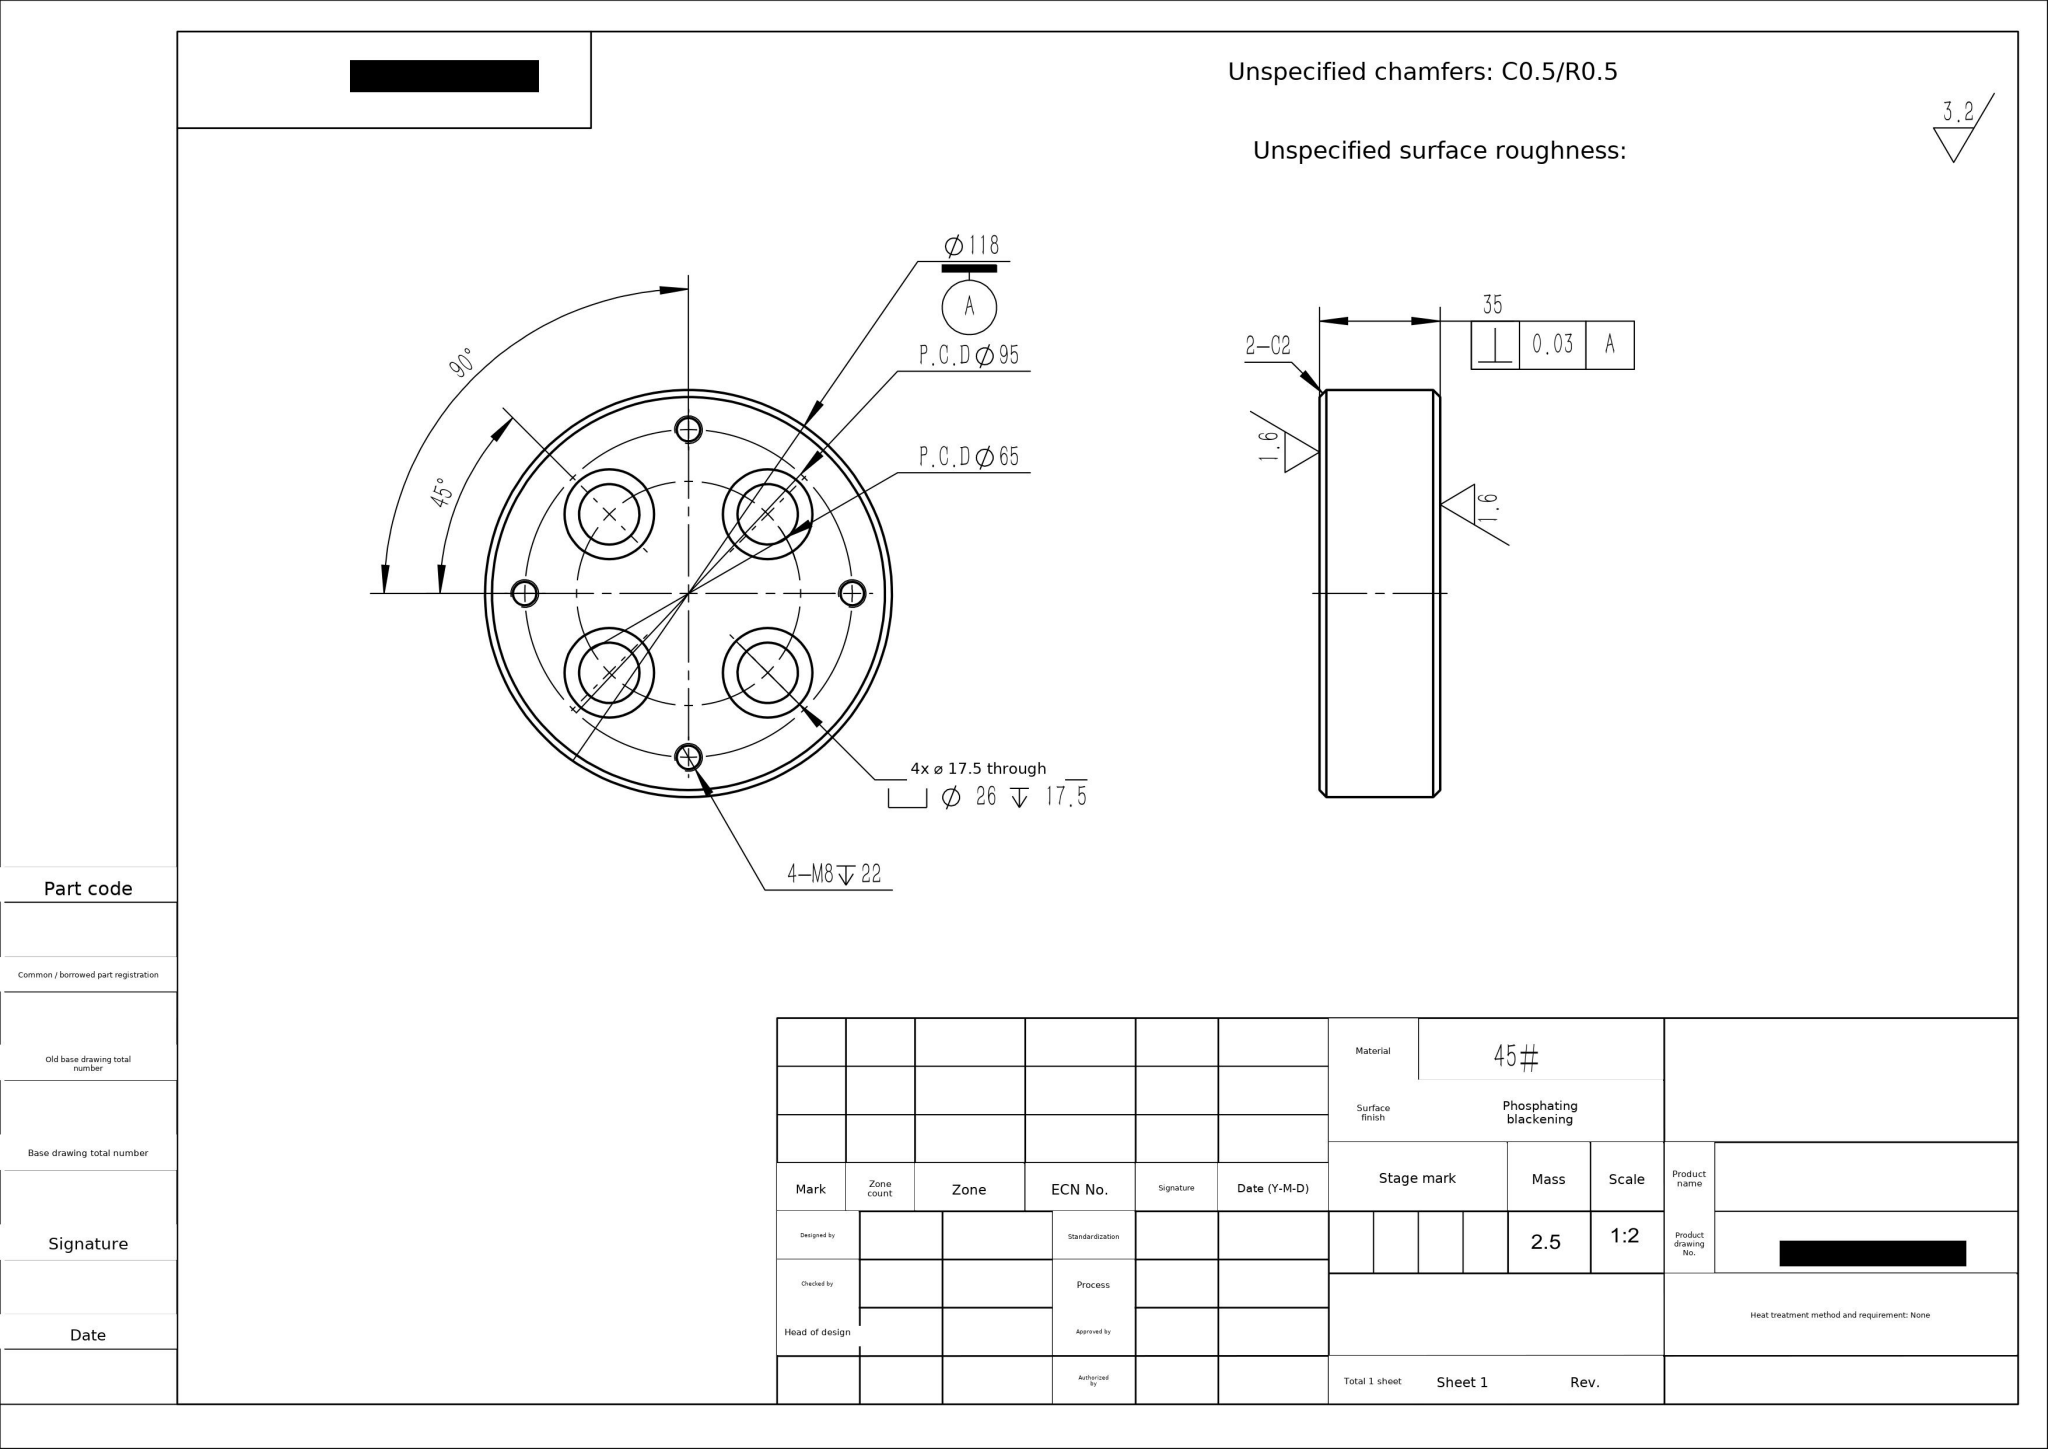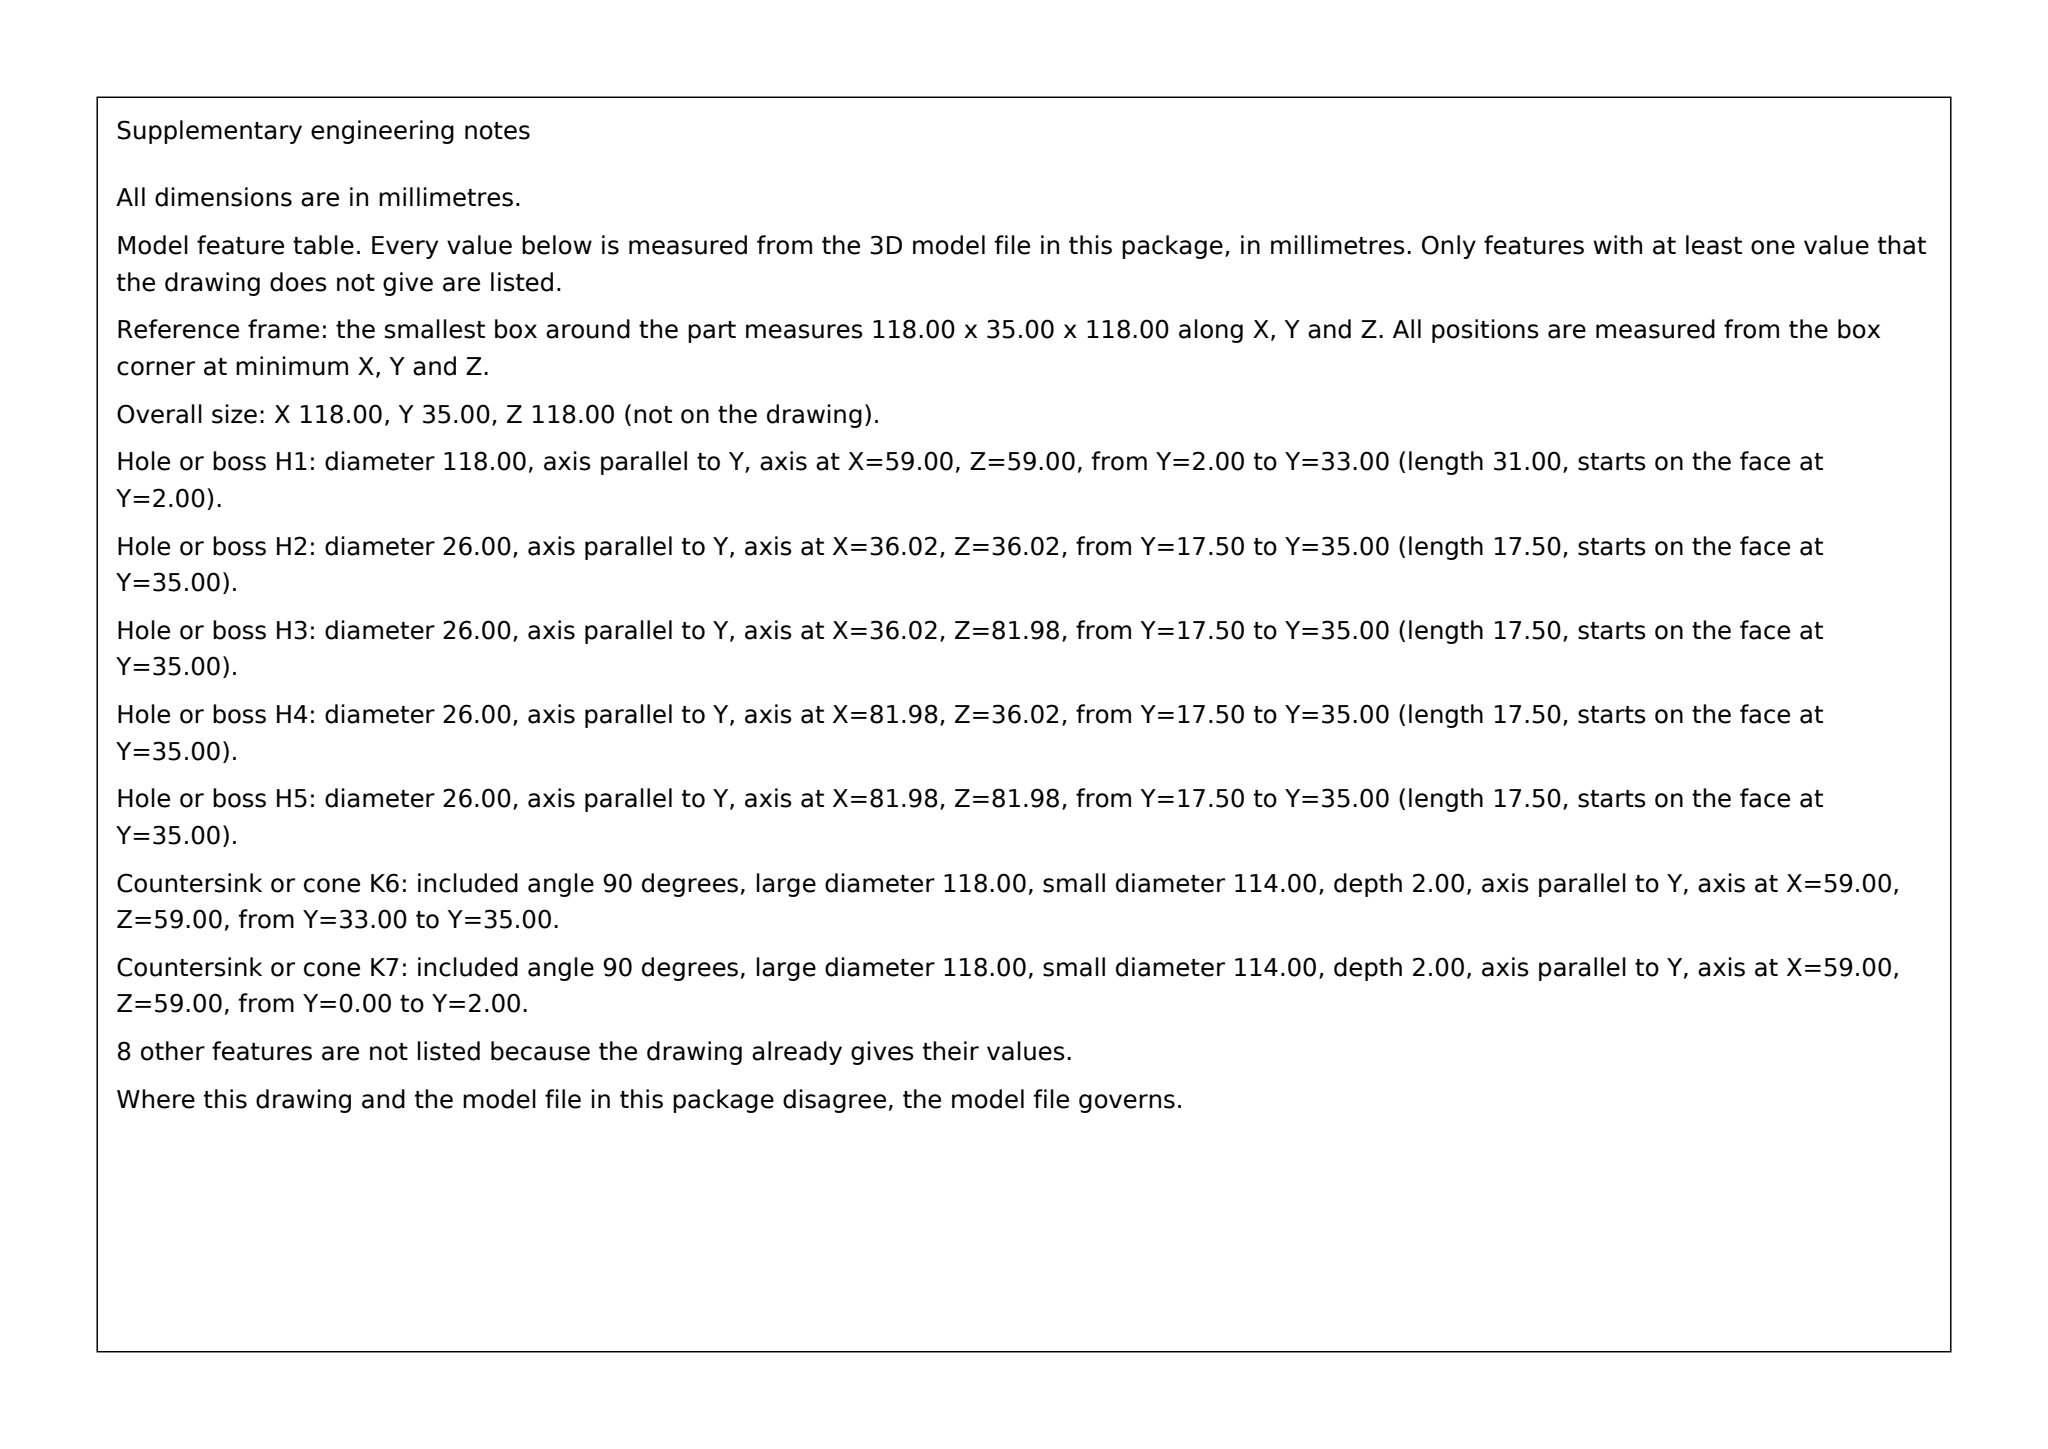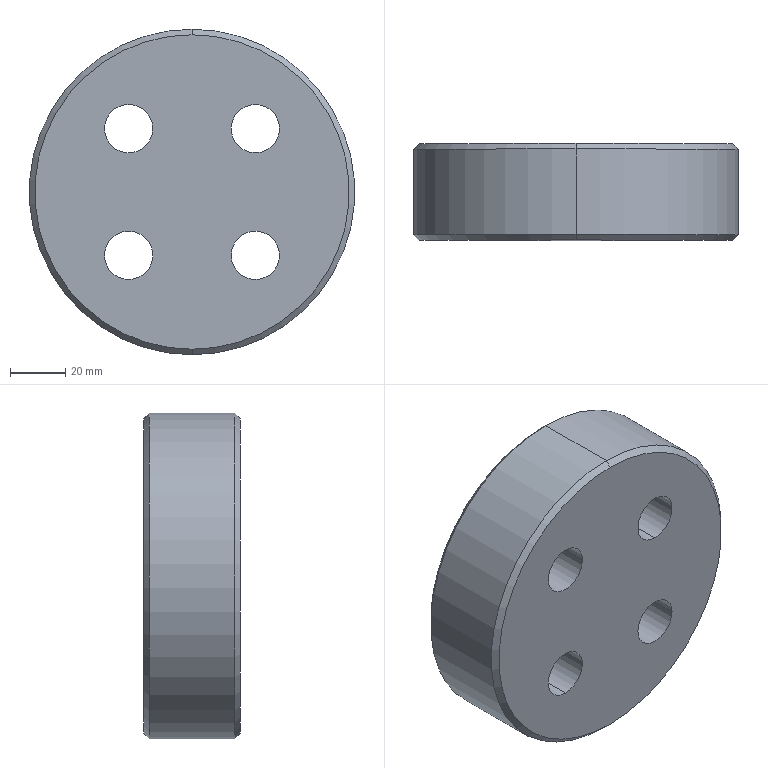Part | SolidWorks | mm | material 45# | 1 solid | 44 faces | box 118 x 35 x 118 mm | volume 324284 mm3 | cylinder 26 | cone 12 | plane 6 | commonest cylinder face diameters 26 x8 17.5 x8 6.8 x8 118 x2
build123d program:
from build123d import *

# Parameters (mm, degrees)
SKETCH1_R           = 59
BOSS_EXTRUDE1_DEPTH = 35
CIRPATTERN1_COUNT   = 4
CIRPATTERN2_COUNT   = 4
CHAMFER1_SIZE       = 2


with BuildPart() as part:
    # Sketch1 → Boss-Extrude1 (new body)
    with BuildSketch(Plane(origin=(0, 0, 0), x_dir=(1, 0, 0), z_dir=(0, 1, 0))):
        with Locations(Location((0, 0, 0), (0, 0, 270))):
            Circle(SKETCH1_R)
    extrude(amount=BOSS_EXTRUDE1_DEPTH)

    # Sketch3 → M8 Tapped Hole1 (revolve, cut)
    with BuildSketch(Plane(origin=(0, 35, -47.5), x_dir=(0, 0, 1), z_dir=(1, 0, 0))):
        Polygon((0, 0), (0, 22.043), (3.4, 20), (3.4, 0), align=None)
    m8_tapped_hole1 = revolve(axis=Axis((0, 41.35, -47.5), (0, -1, 0)), mode=Mode.SUBTRACT)

    # CirPattern1: M8 Tapped Hole1 ×4 about axis
    cirpattern1_axis = Axis((0, 0, 0), (0, 1, 0))
    for i in range(1, CIRPATTERN1_COUNT):
        add(m8_tapped_hole1.rotate(cirpattern1_axis, i * 360 / CIRPATTERN1_COUNT), mode=Mode.SUBTRACT)

    # Sketch5 → Hole Size_According to_Type 1 of Hexagon (revolve, cut)
    with BuildSketch(Plane(origin=(-22.981, 35, -22.981), x_dir=(0, 0, 1), z_dir=(1, 0, 0))):
        Polygon((0, 0), (0, 43.258), (8.75, 38), (8.75, 17.5), (13, 17.5), (13, 0), align=None)
    hole_size_according_to_type_1_of_hexagon = revolve(axis=Axis((-22.981, 41.35, -22.981), (0, -1, 0)), mode=Mode.SUBTRACT)

    # CirPattern2: Hole Size_According to_Type 1 of Hexagon ×4 about axis
    cirpattern2_axis = Axis((0, 0, 0), (0, 1, 0))
    for i in range(1, CIRPATTERN2_COUNT):
        add(hole_size_according_to_type_1_of_hexagon.rotate(cirpattern2_axis, i * 360 / CIRPATTERN2_COUNT), mode=Mode.SUBTRACT)

    # Chamfer1
    chamfer1_edges = [part.edges().sort_by_distance(p)[0] for p in [
        (0, 0, -59),
        (0, 35, -59),
    ]]
    chamfer(chamfer1_edges, length=CHAMFER1_SIZE)


solid = part.part